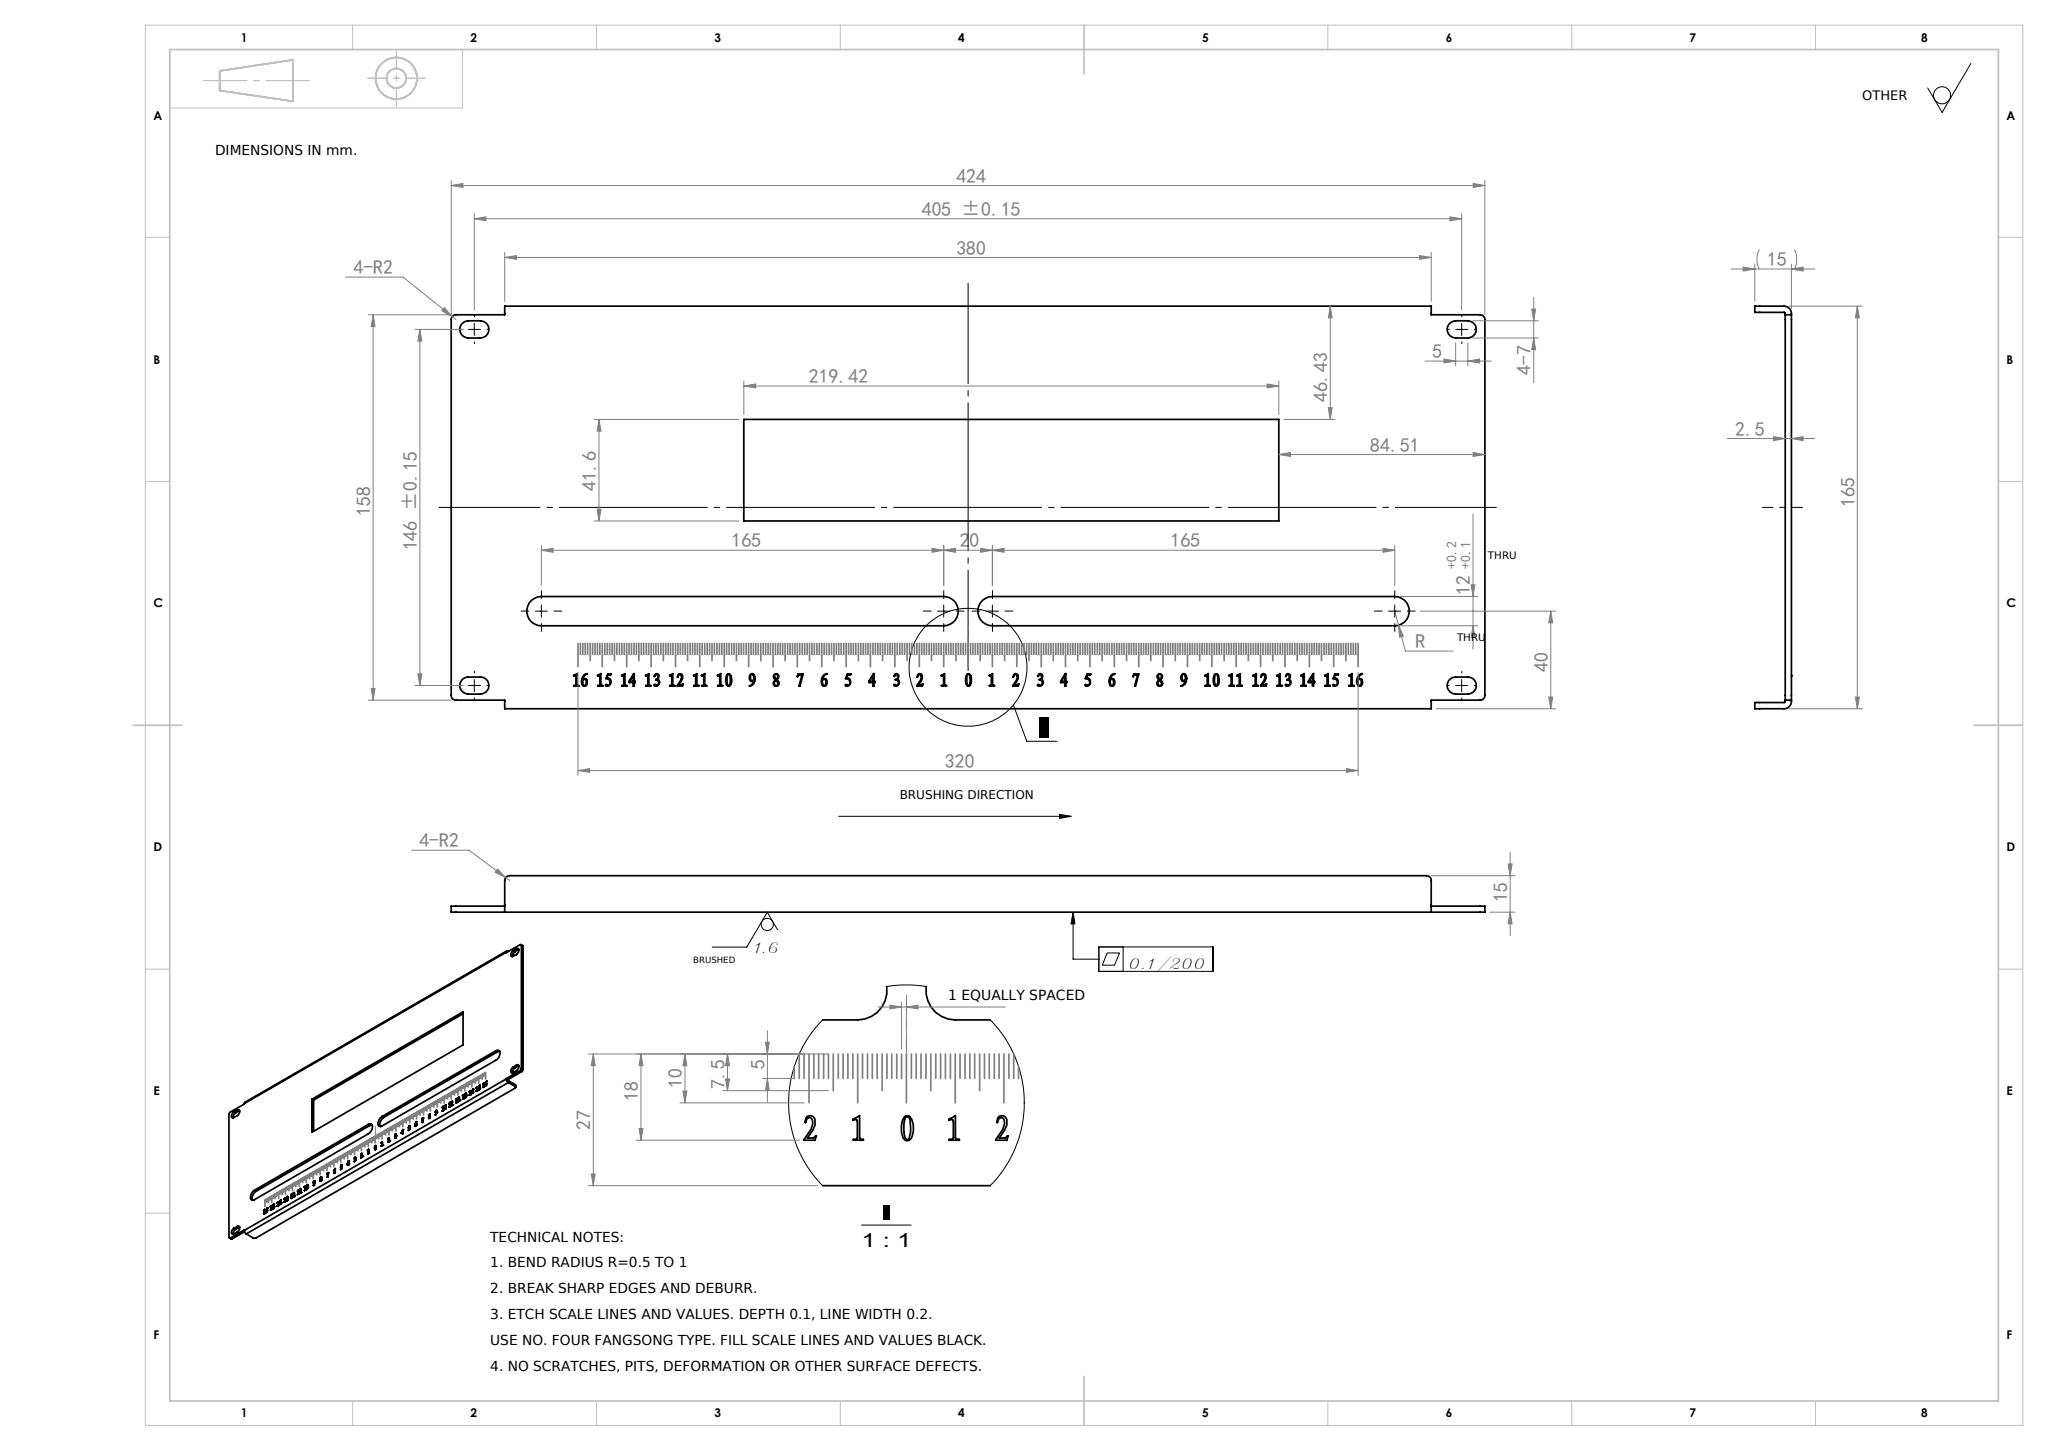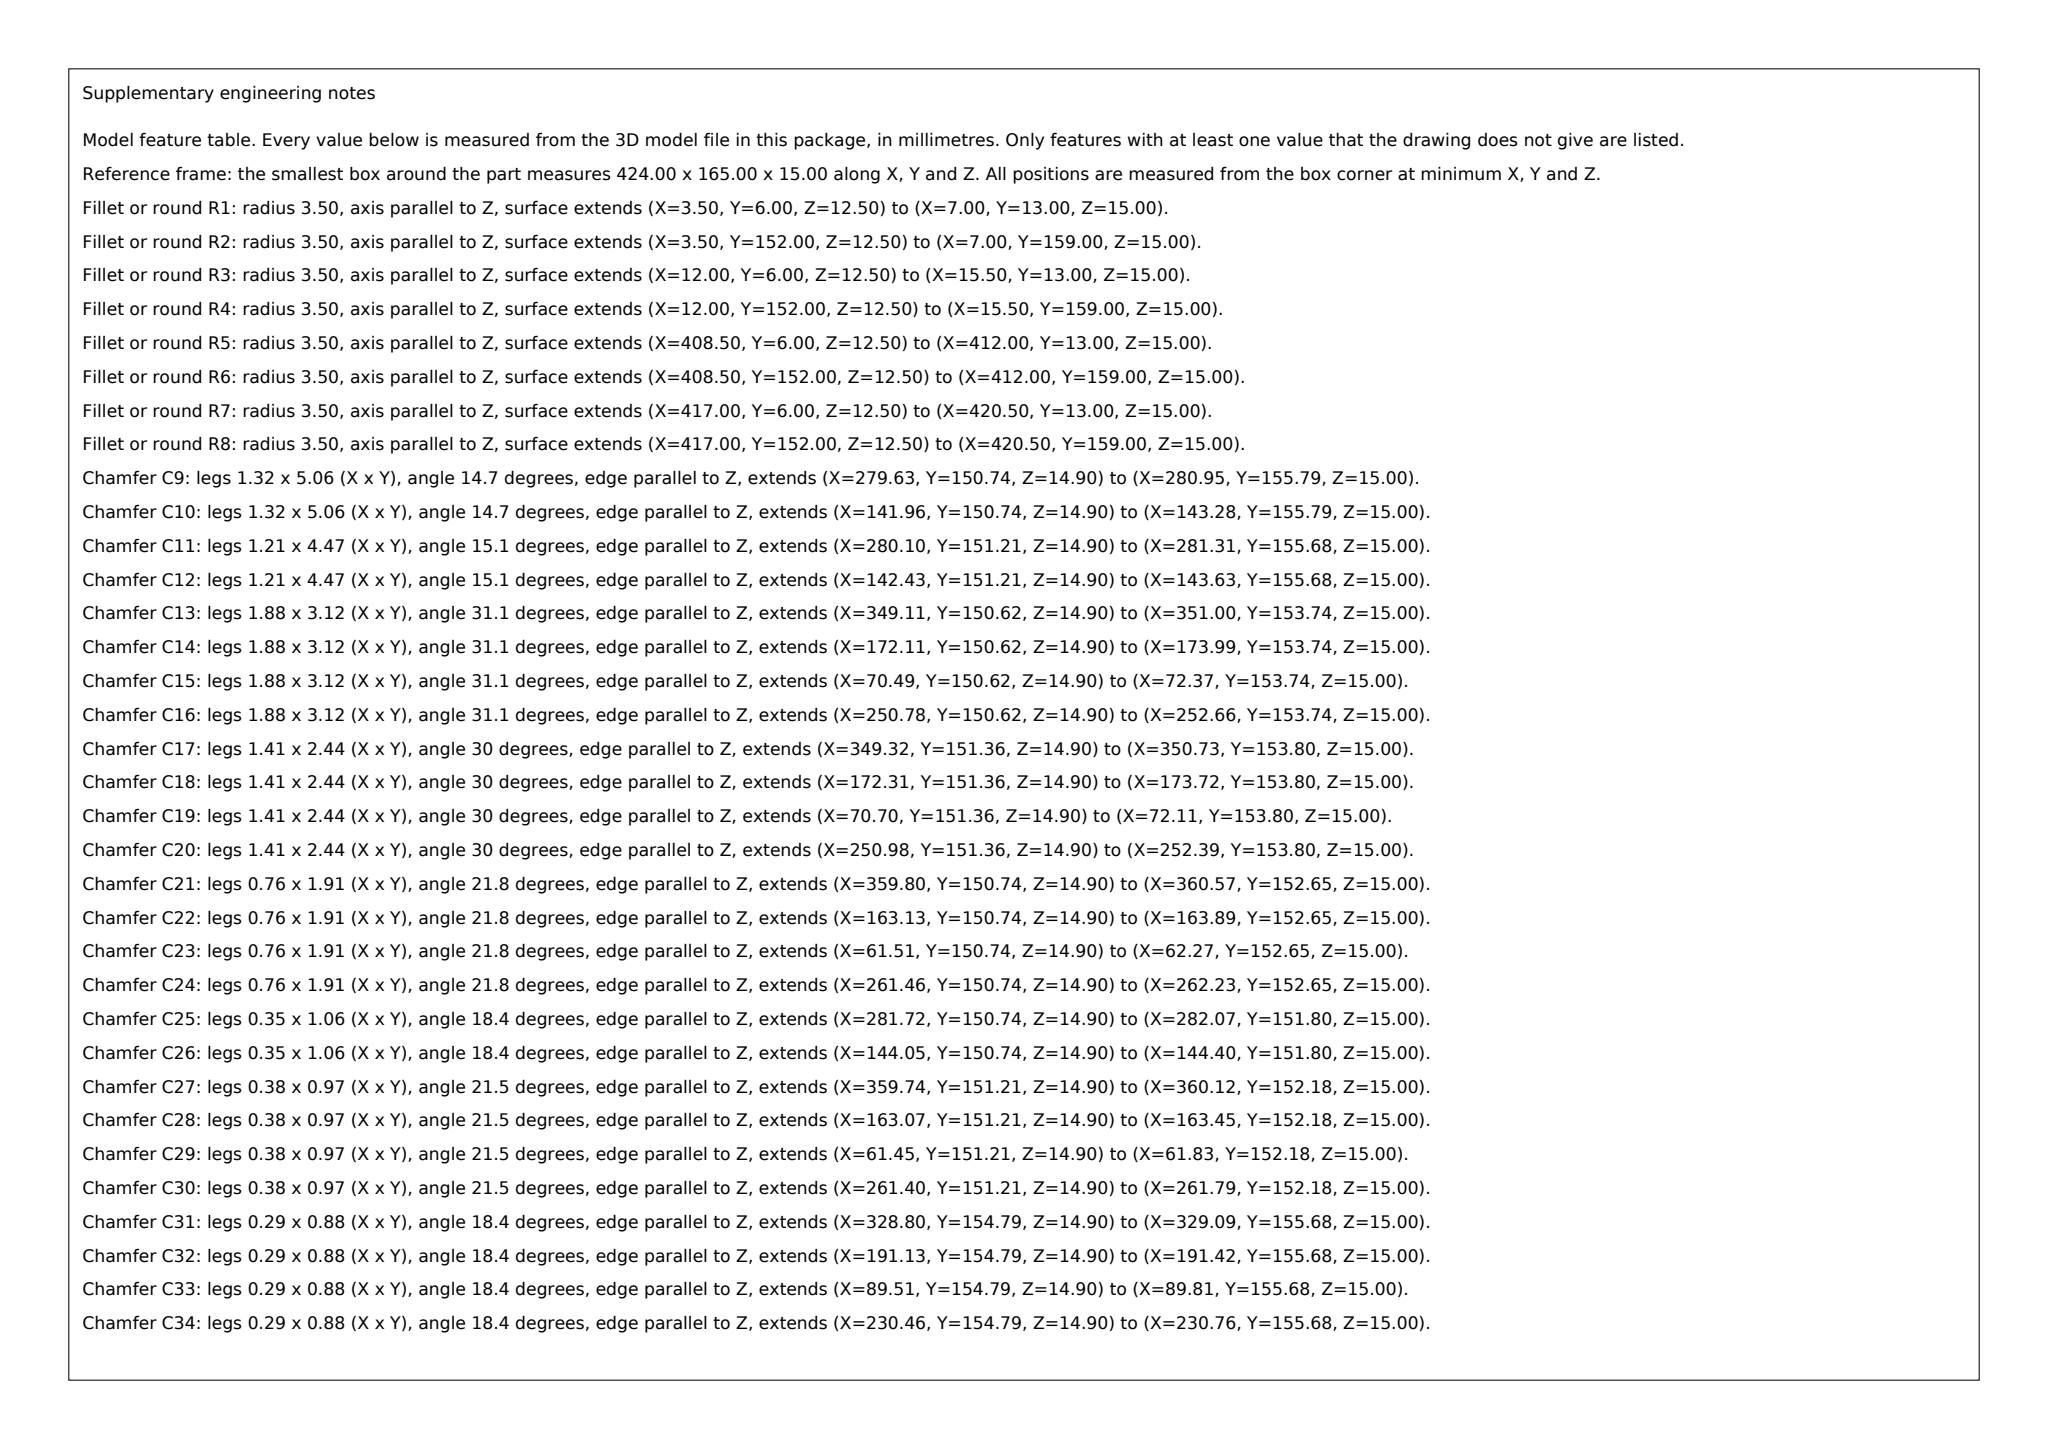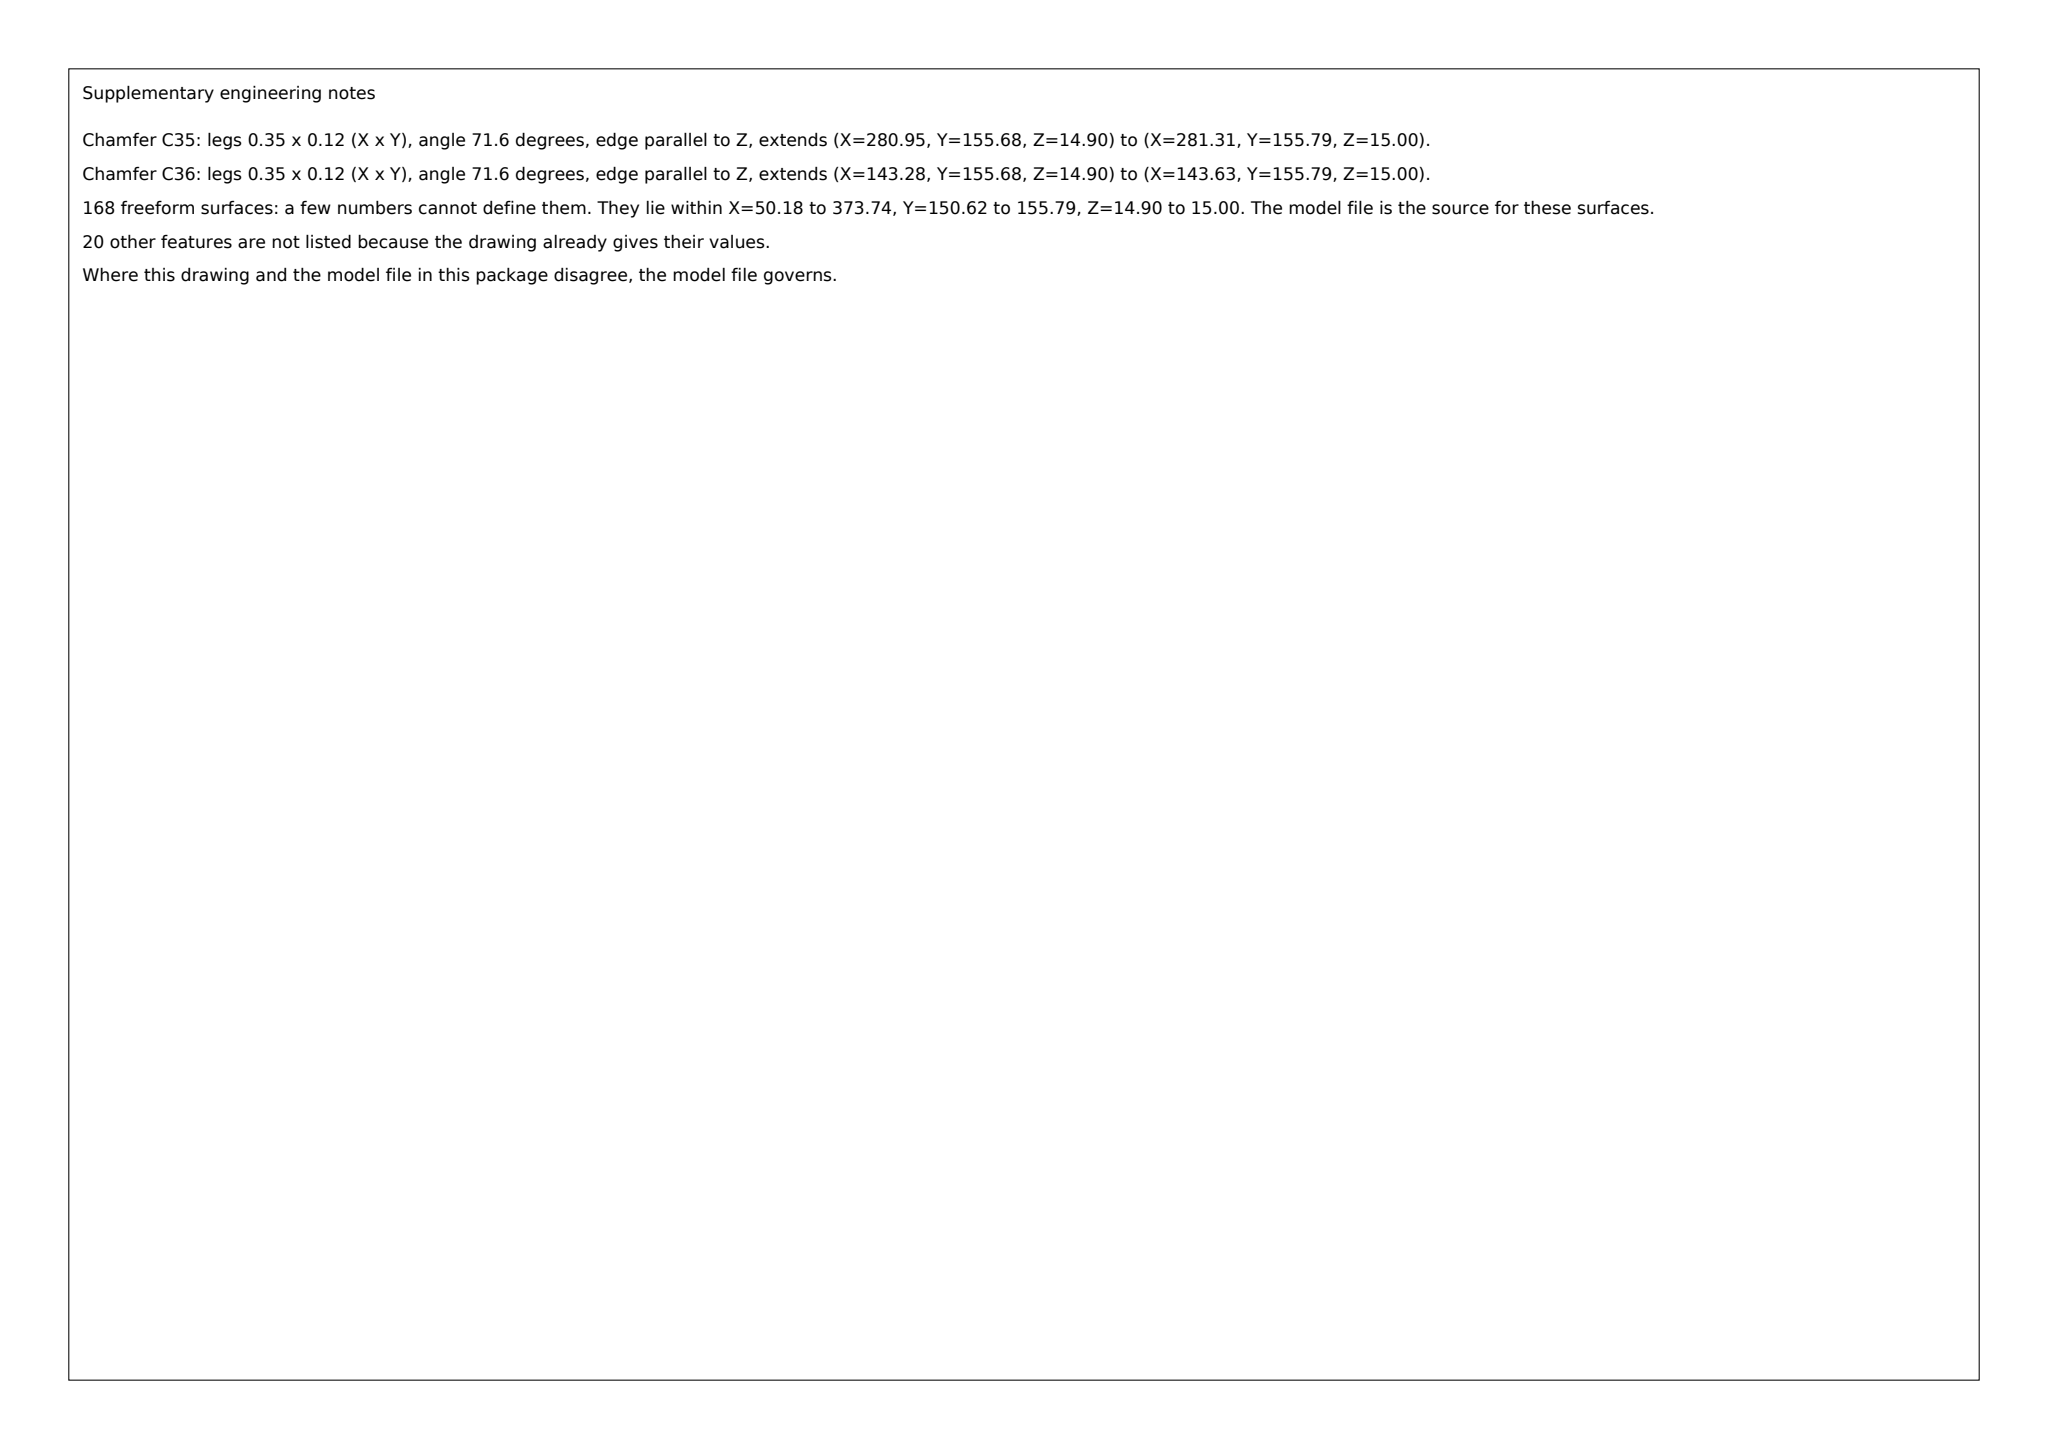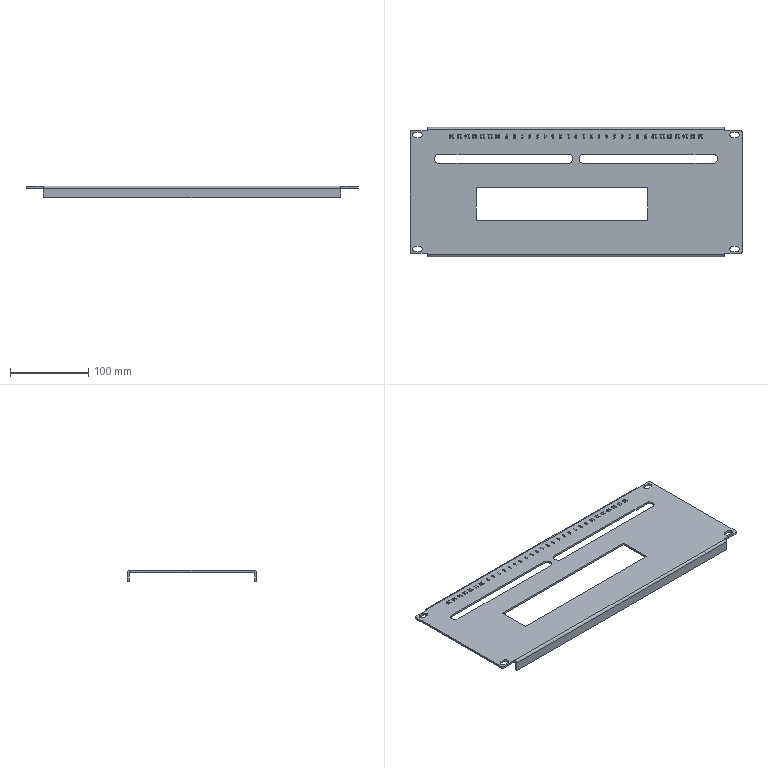Part | SolidWorks | mm | 1 solid | 532 faces | box 424 x 165 x 15 mm | volume 162398 mm3 | plane 334 | spline 168 | cylinder 30 | commonest cylinder face diameters 7 x12 4 x8 12 x6 6 x2 1 x2